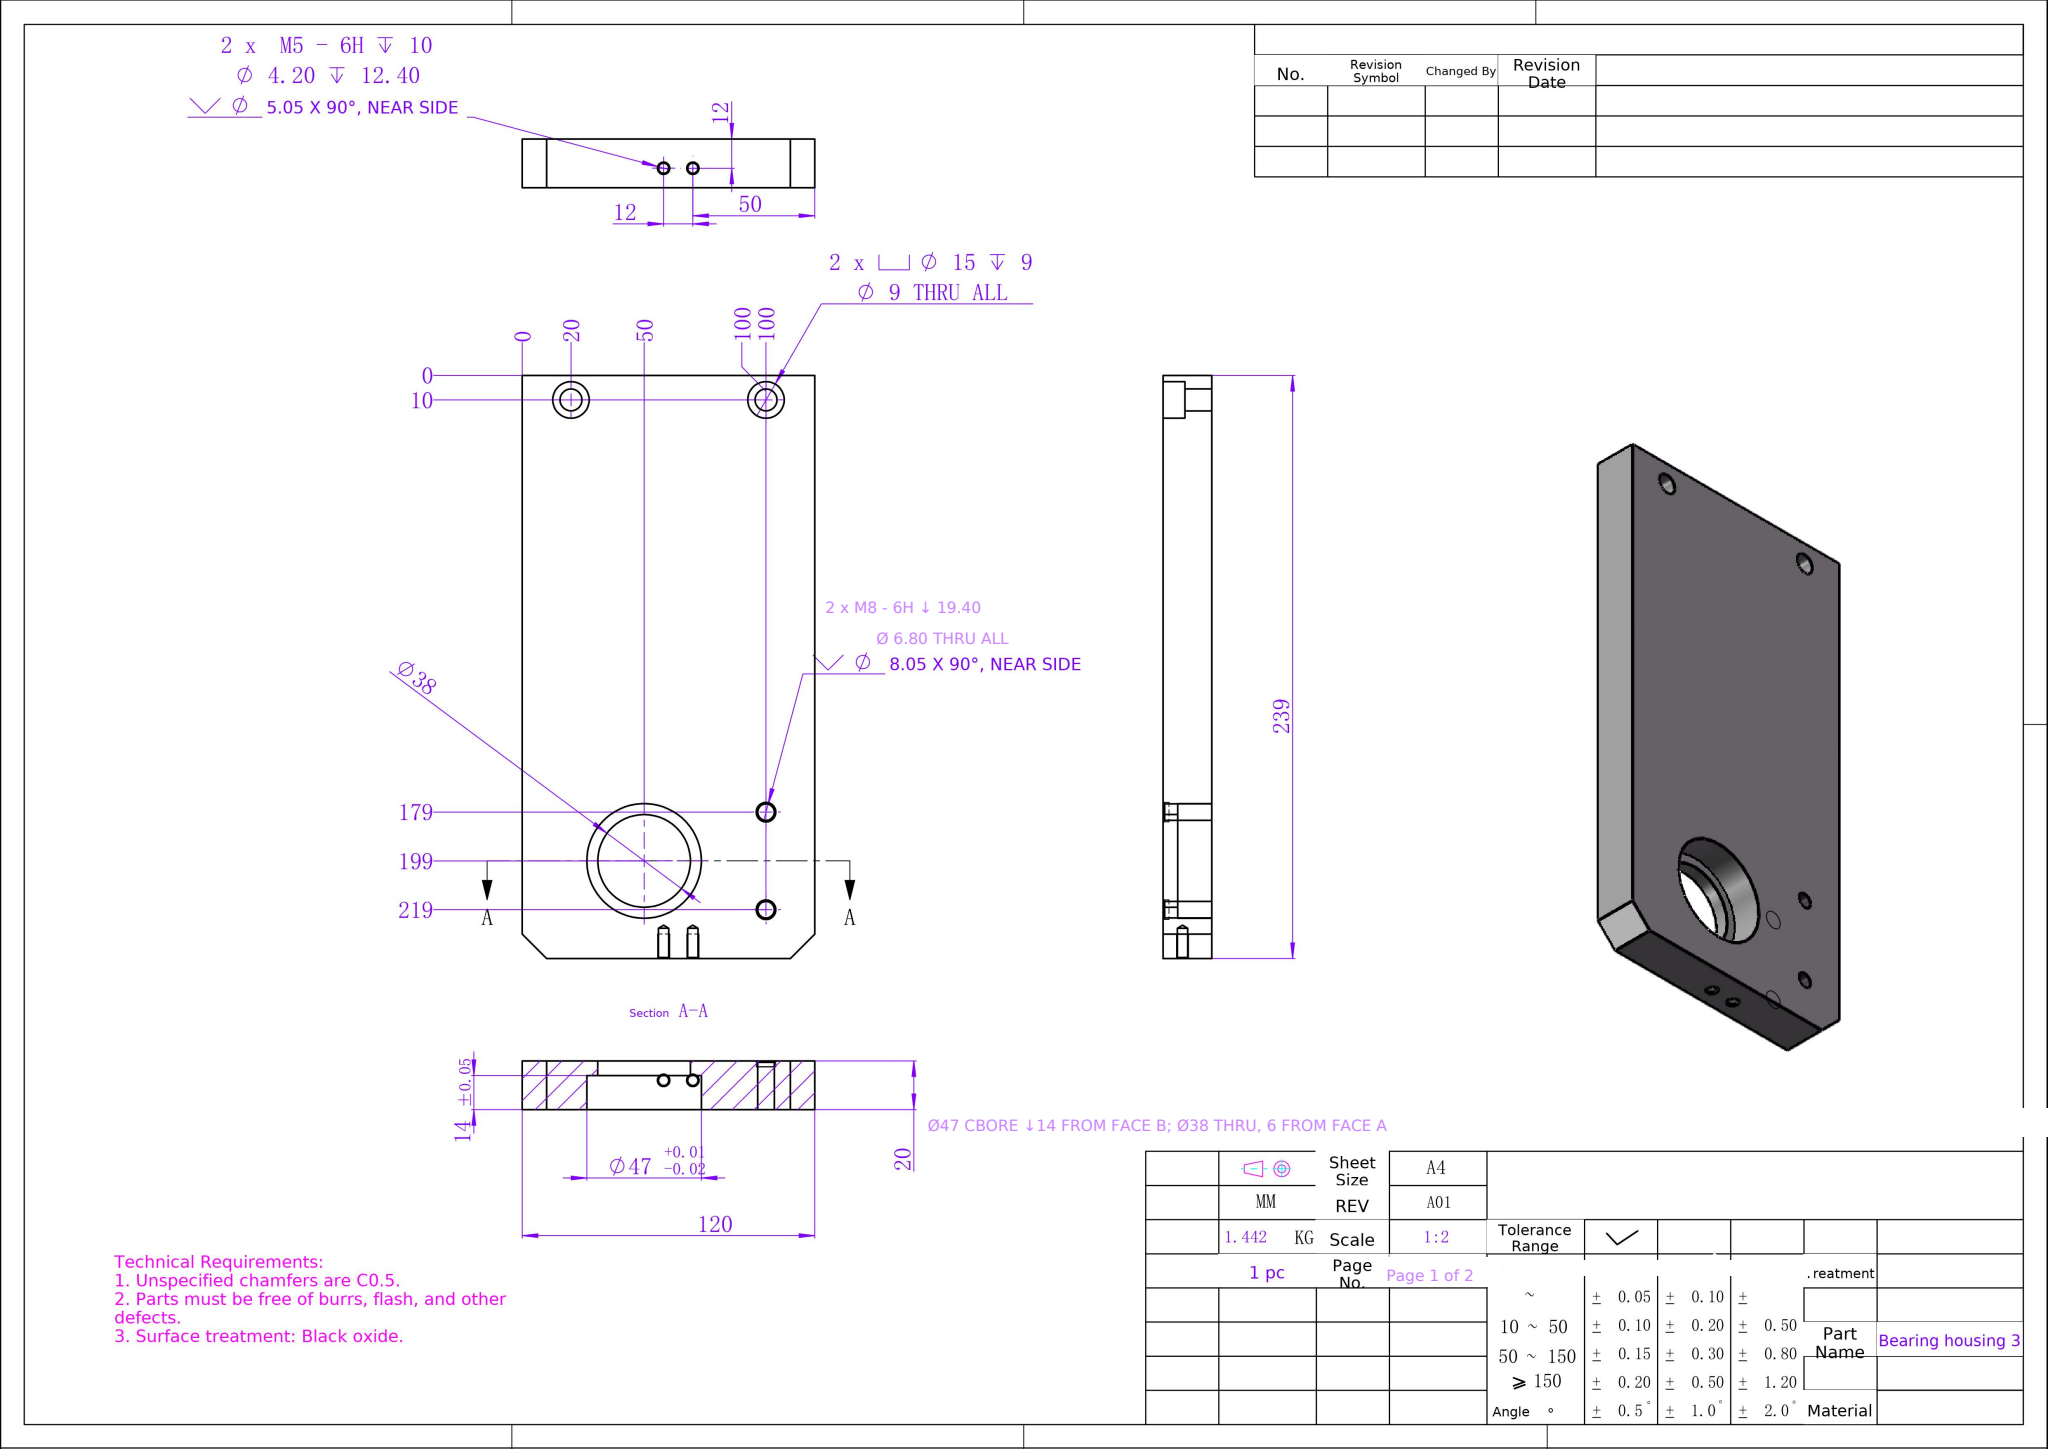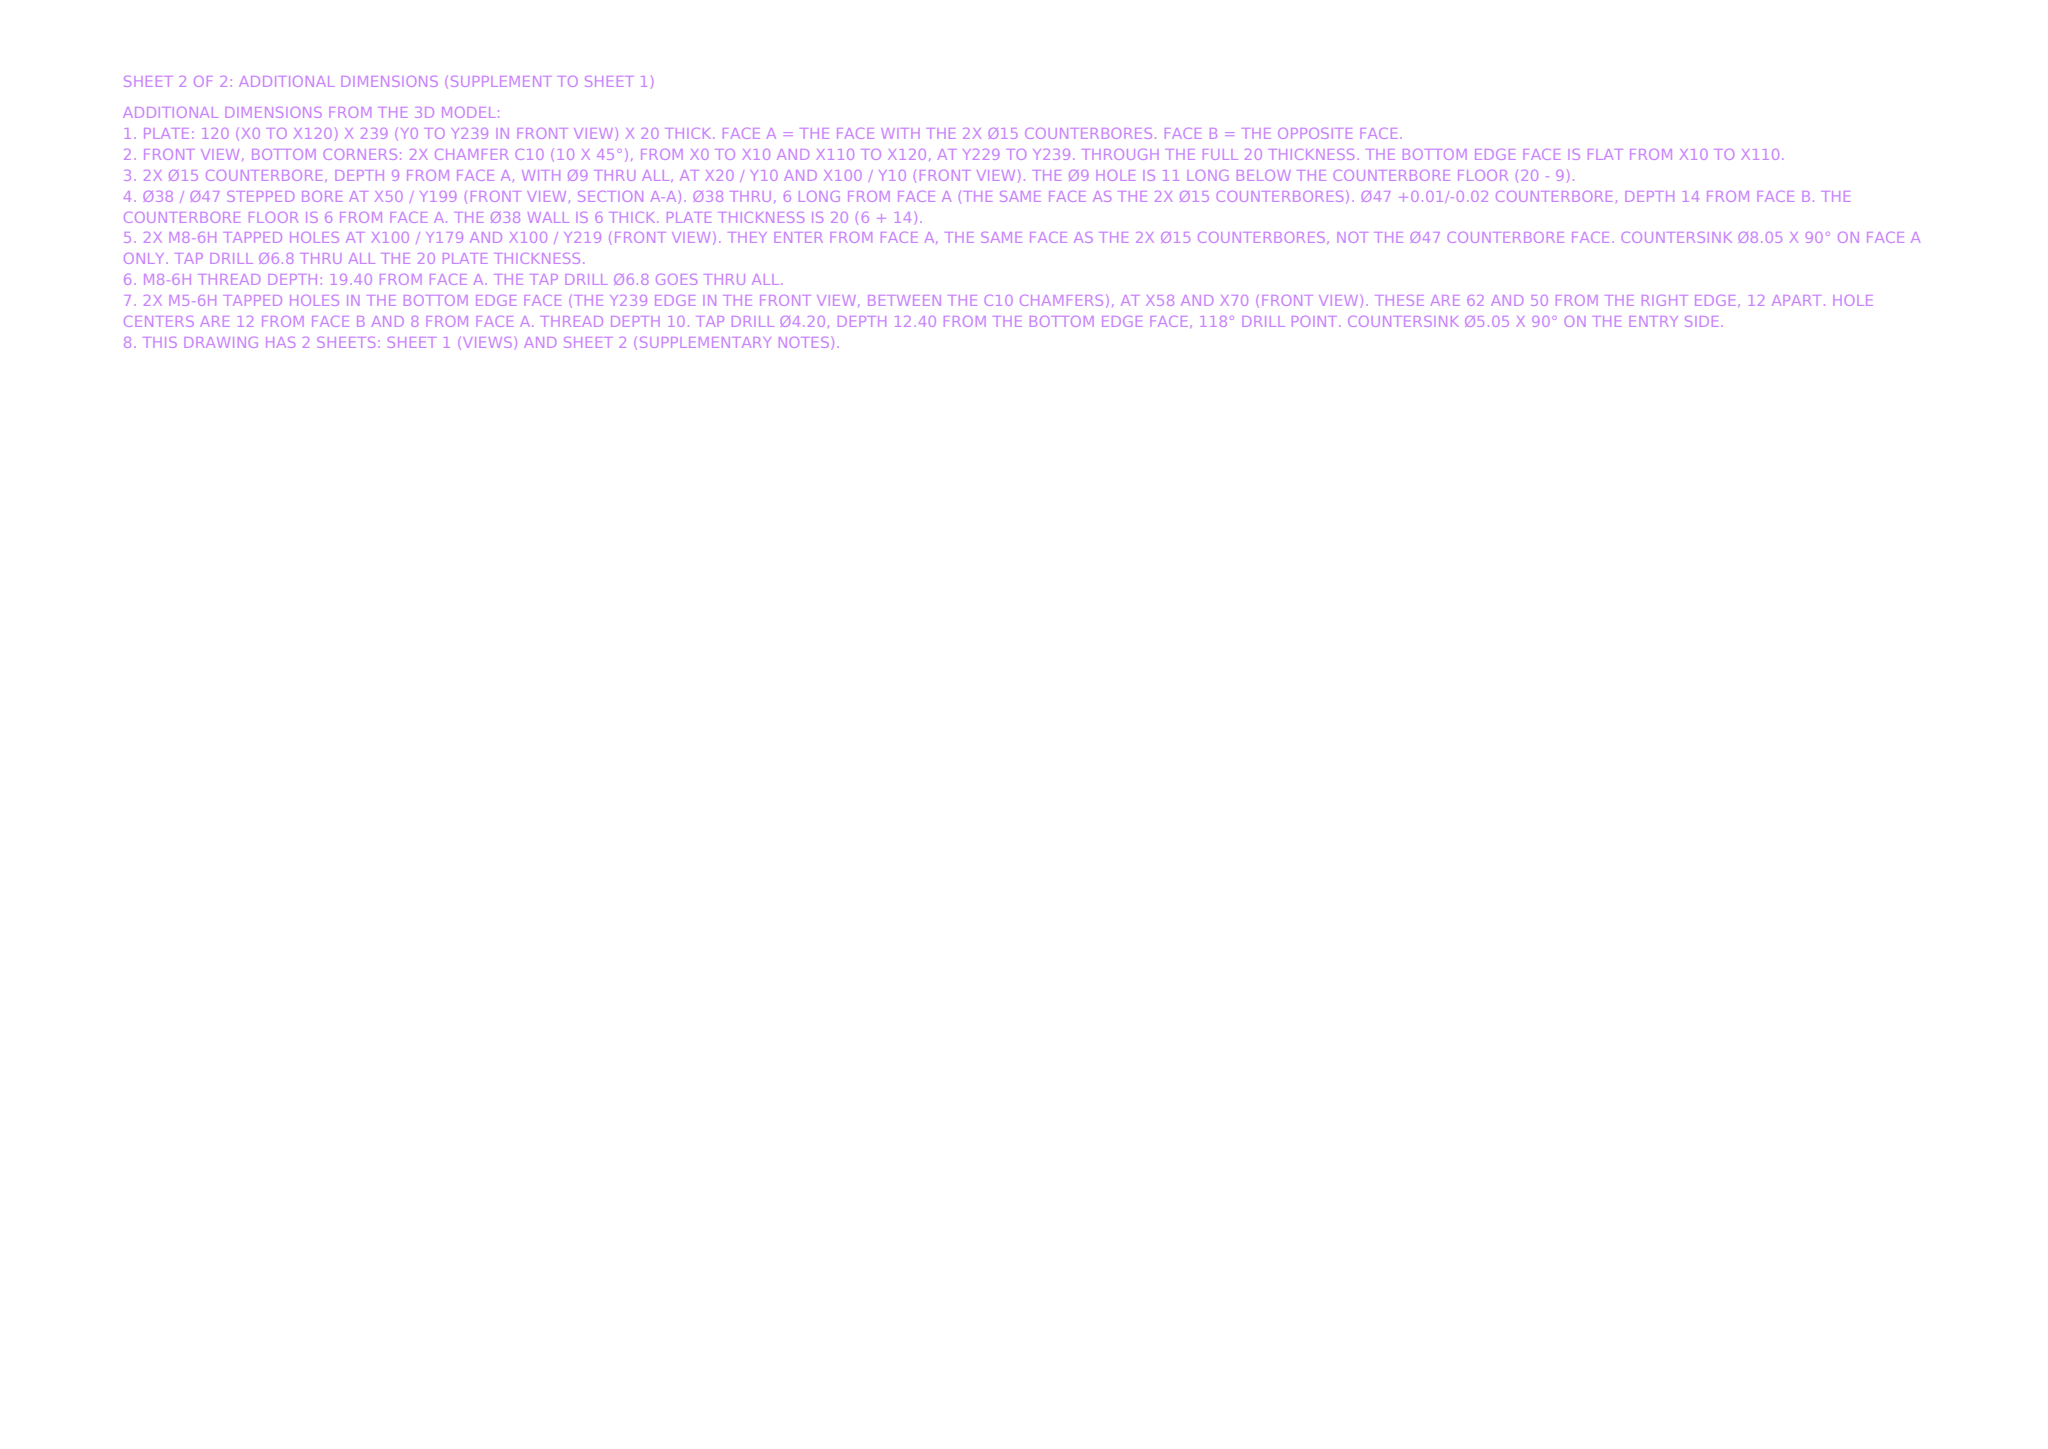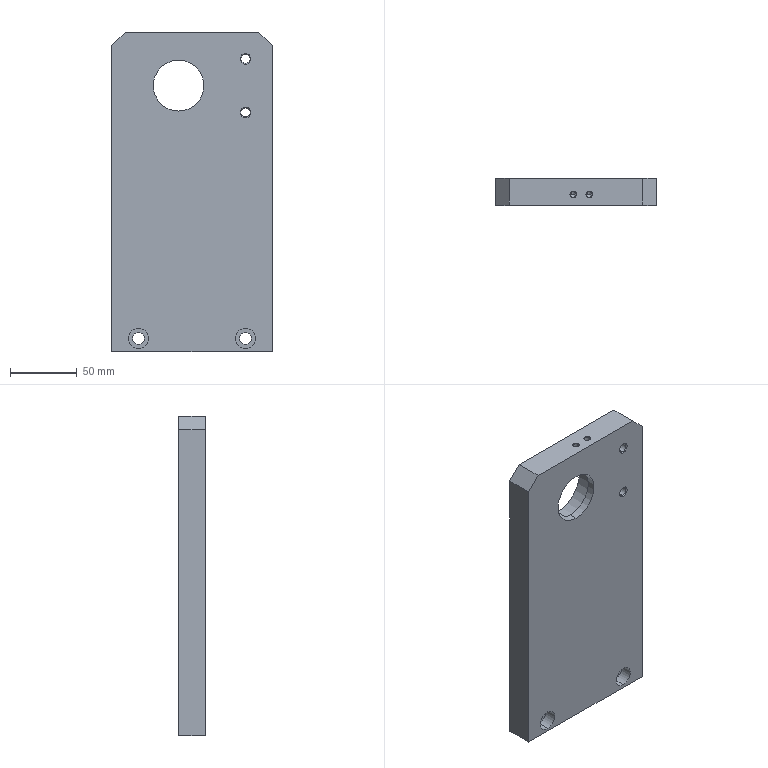Part | NX | mm | 1 solid | 43 faces | box 120 x 20 x 239 mm | volume 534106 mm3 | cylinder 20 | cone 12 | plane 11 | commonest cylinder face diameters 4.2 x4 6.8 x4 9 x4 15 x4 38 x2 47 x2